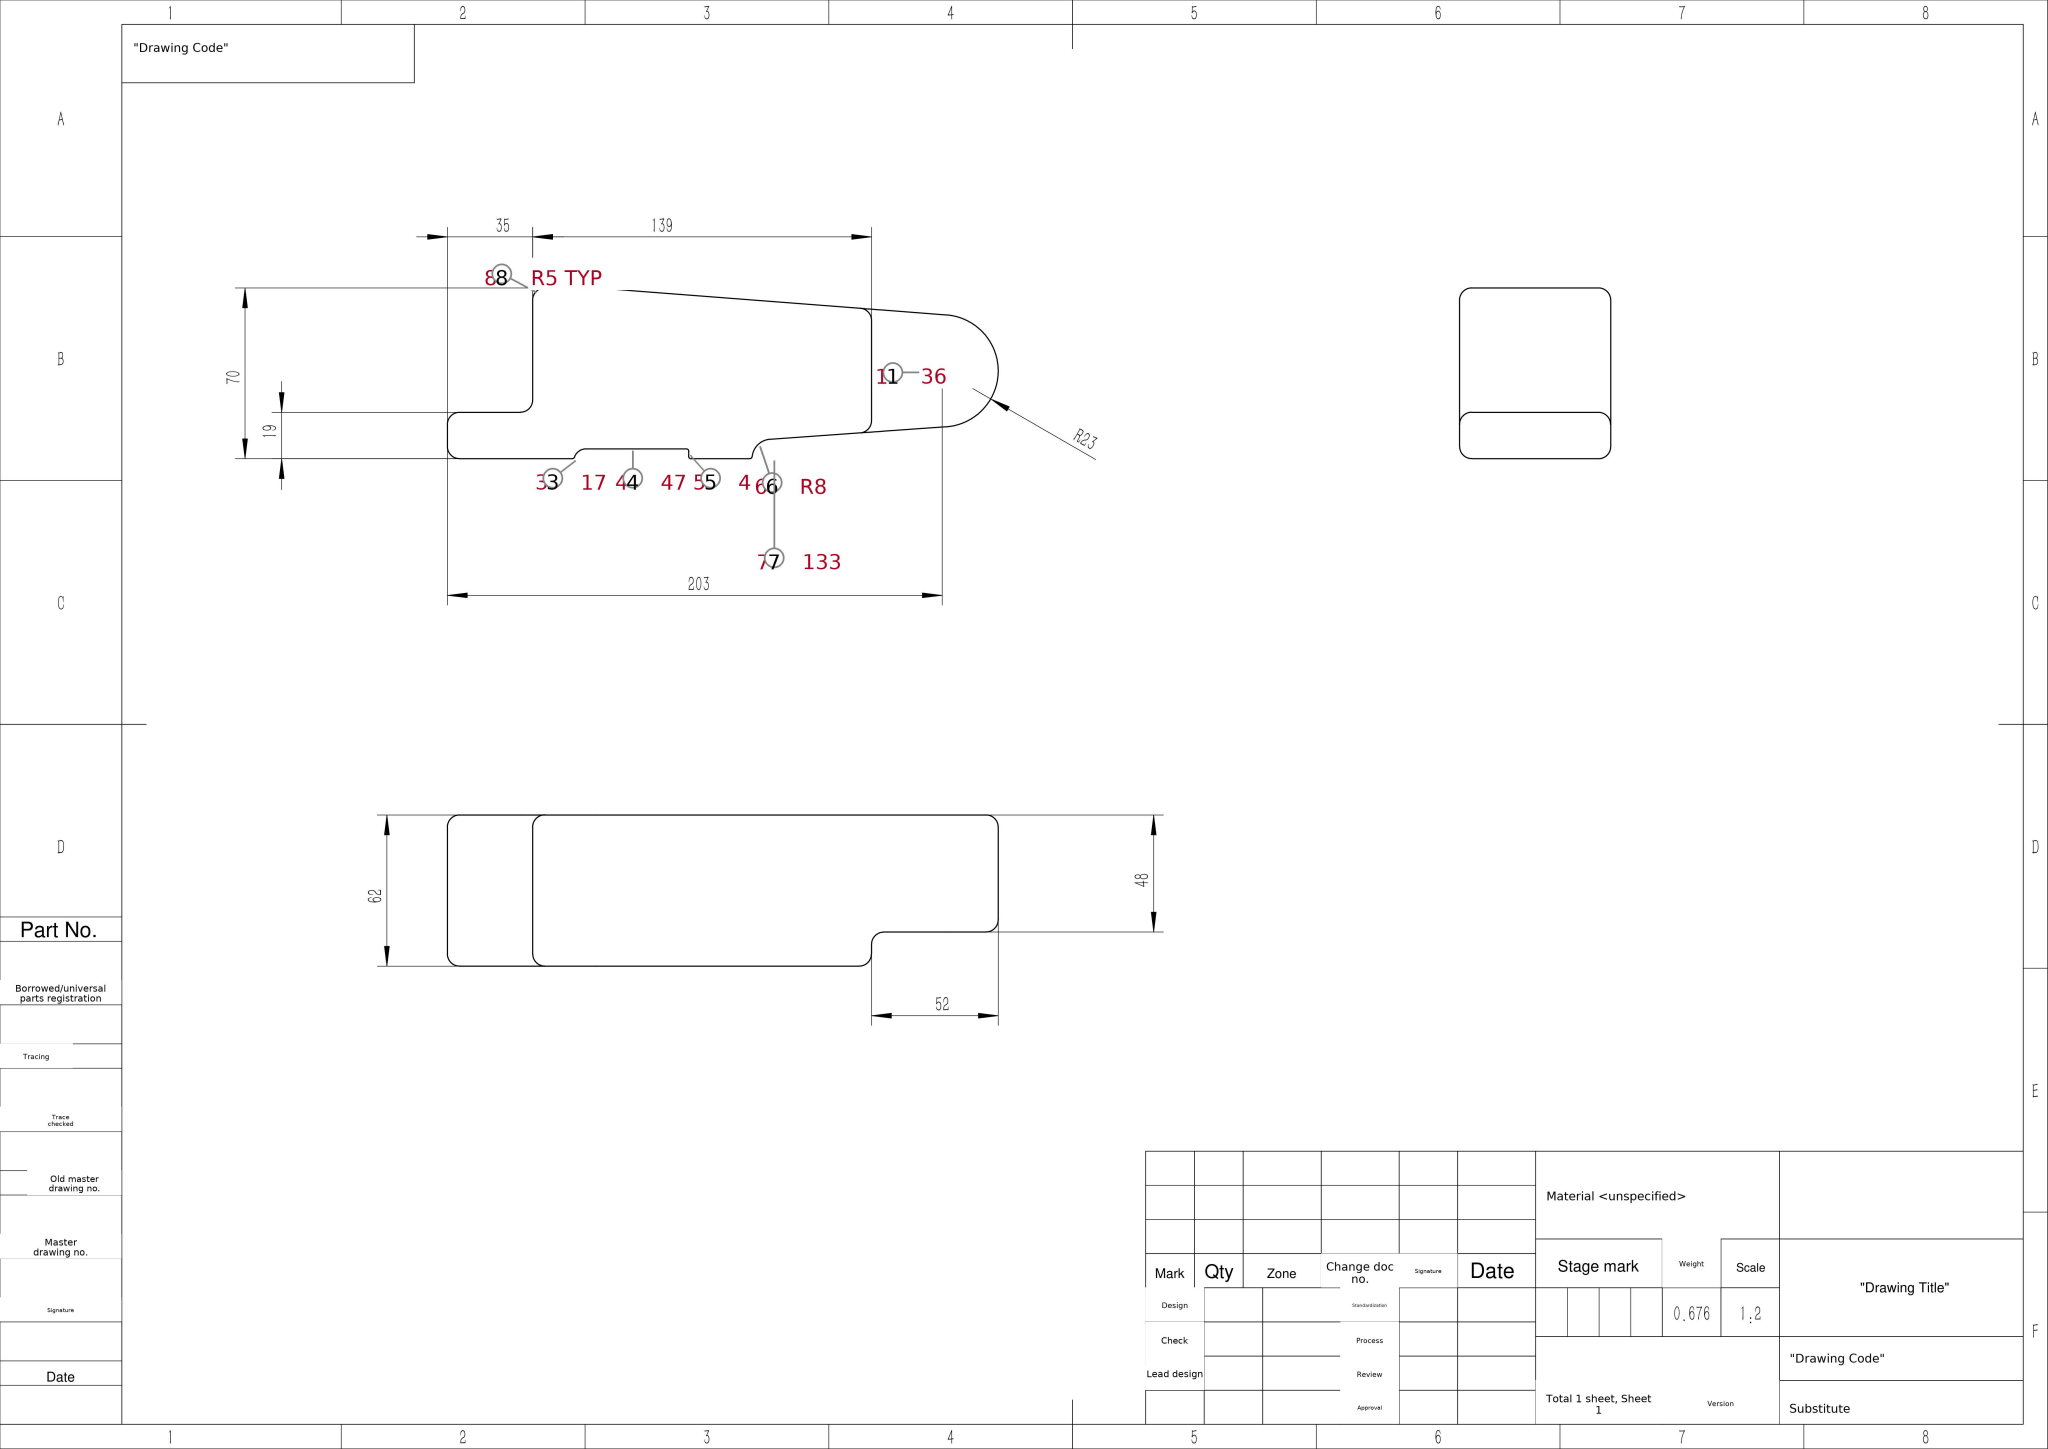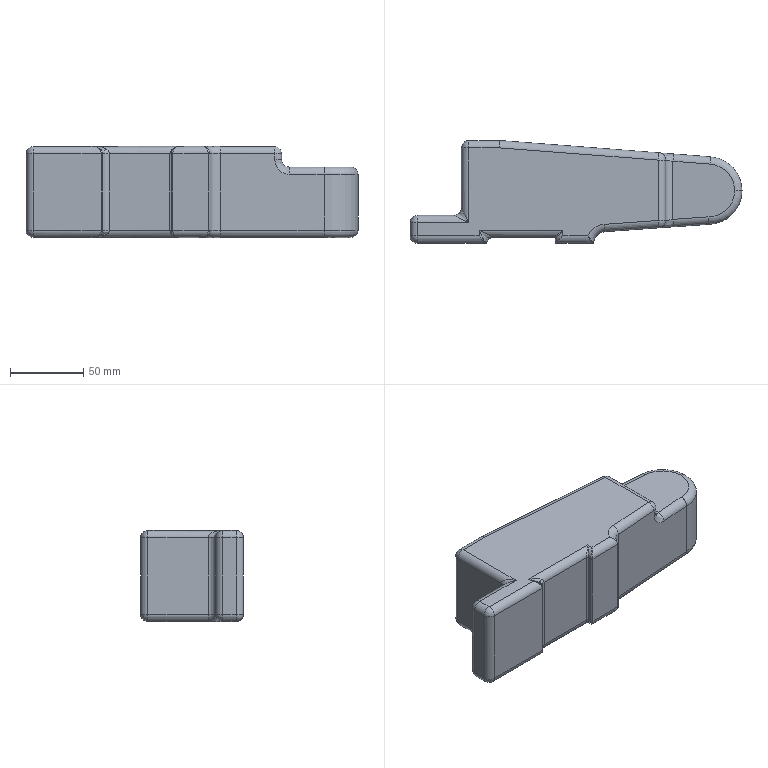Part | SolidWorks | mm | 1 solid | 93 faces | box 226 x 70 x 62 mm | volume 675799 mm3 | cylinder 41 | spline 23 | plane 14 | sphere 8 | torus 7 | commonest cylinder face diameters 10 x33 2 x6 46 x1 16 x1